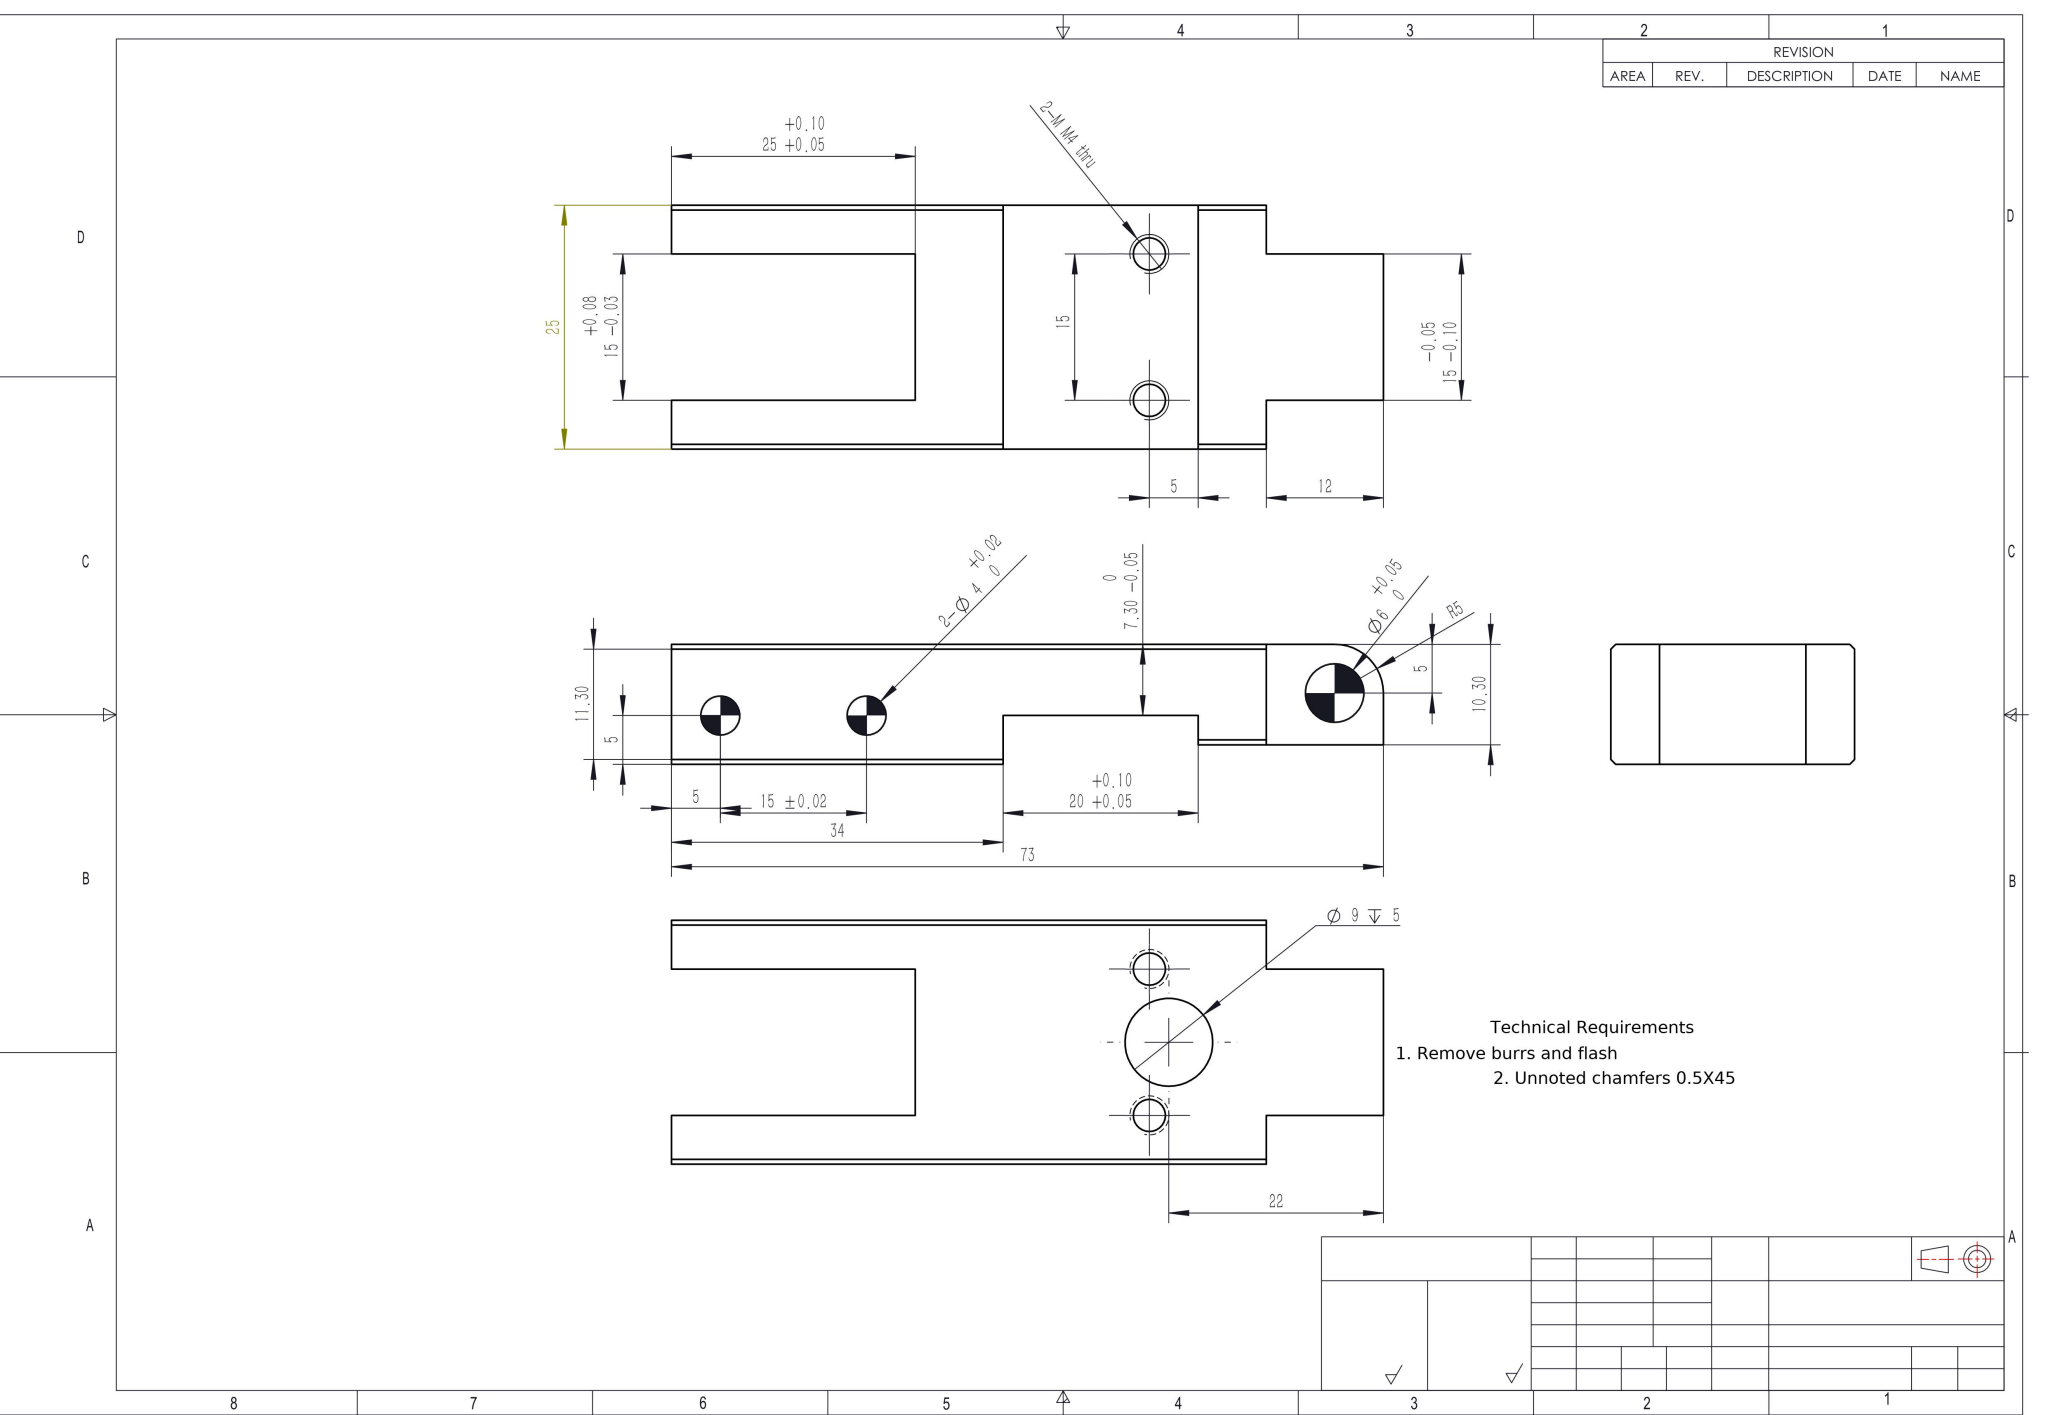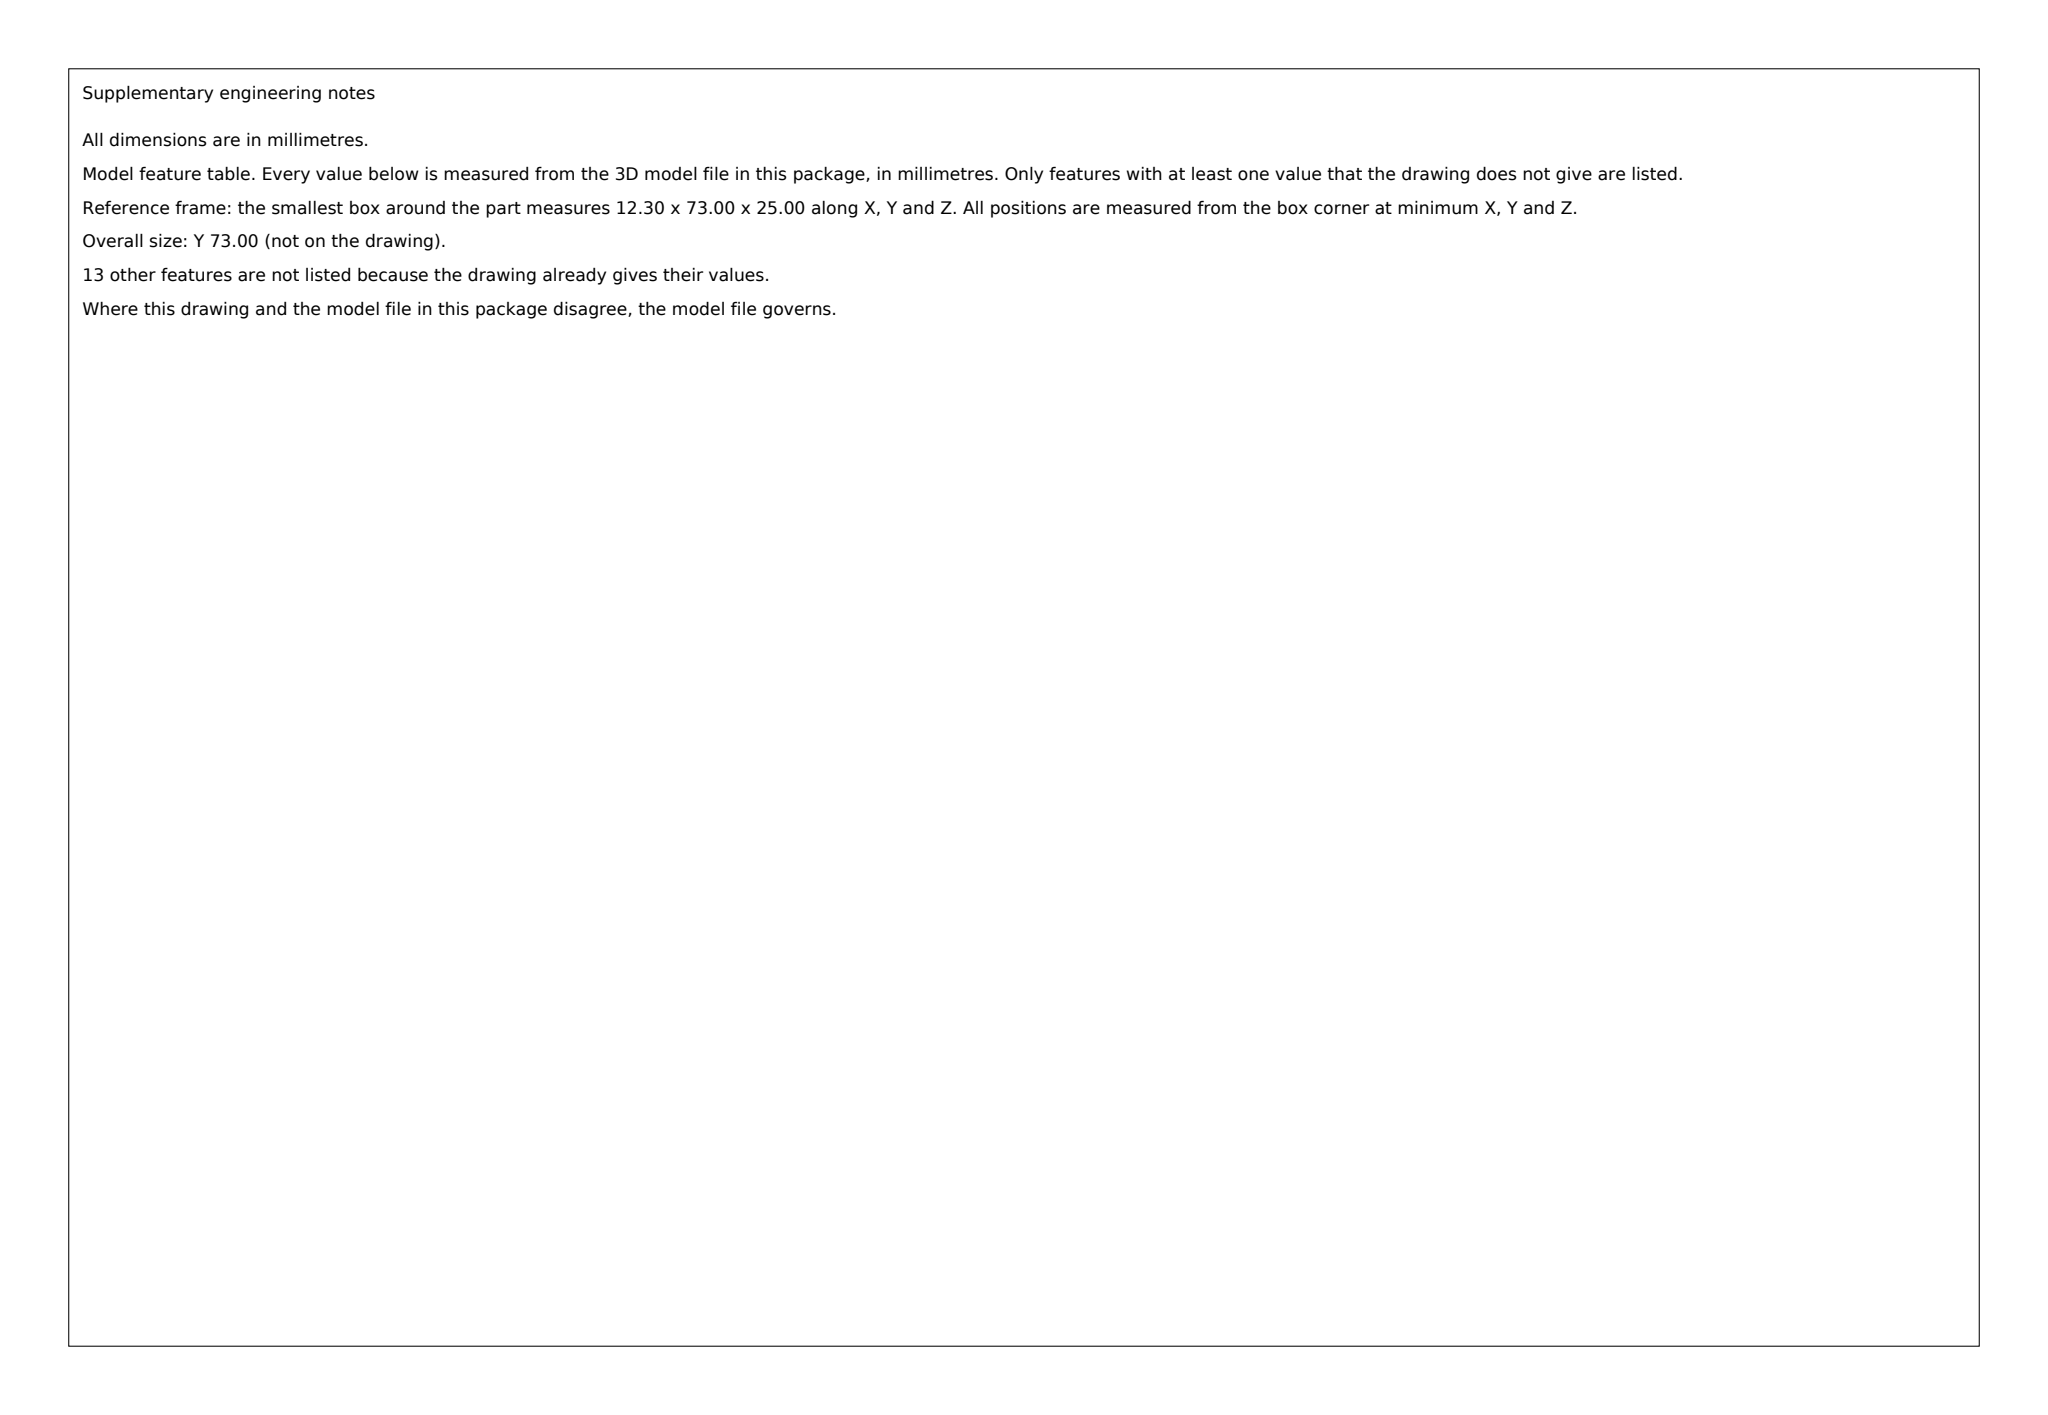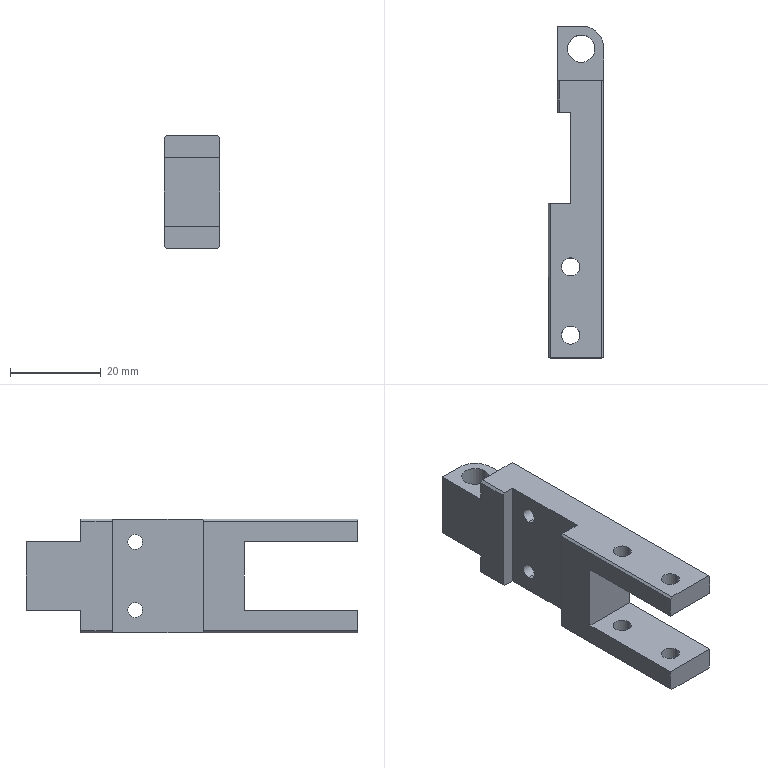Part | SolidWorks | mm | 1 solid | 42 faces | box 12.3 x 73 x 25 mm | volume 11925 mm3 | plane 25 | cylinder 17 | commonest cylinder face diameters 4 x8 3.3 x4 9 x2 6 x2 10 x1
build123d program:
from build123d import *

# Parameters (mm, degrees)
SKETCH1_W                    = 12.3
SKETCH1_H                    = 25
BOSS_EXTRUDE1_DEPTH          = 85
SKETCH2_W                    = 25
SKETCH2_H                    = 5
BOSS_EXTRUDE2_DEPTH          = 5
SKETCH4_W                    = 15
SKETCH4_H                    = 35
CUT_EXTRUDE1_DEPTH           = 87.79
SIZE_MM_DOWEL_HOLE_1_D       = 4
SKETCH7_W                    = 12.3
SKETCH7_H                    = 10
CUT_EXTRUDE2_DEPTH           = 90.299
SKETCH8_W                    = 5
SKETCH8_H                    = 20
CUT_EXTRUDE3_DEPTH           = 90.299
SKETCH14_W                   = 17.3
SKETCH14_H                   = 5
CUT_EXTRUDE4_DEPTH           = 90.299
SKETCH15_W                   = 12.3
SKETCH15_H                   = 5
CUT_EXTRUDE5_DEPTH           = 9
SKETCH22_W                   = 12.3
SKETCH22_H                   = 15
BOSS_EXTRUDE3_DEPTH          = 3
FILLET1_R                    = 5
SIZE_MM_DOWEL_HOLE_3_D       = 6
SIZE_MM_DOWEL_HOLE_3_DEPTH   = 35
CUT_EXTRUDE7_DEPTH           = 2
F_4_0_4_DIAMETER_HOLE1_D     = 9
F_4_0_4_DIAMETER_HOLE1_DEPTH = 5
M4_TAPPED_HOLE1_D            = 3.3
M4_TAPPED_HOLE1_DEPTH        = 11.5
M4_TAPPED_HOLE1_TIP          = 0.9914
CHAMFER1_SIZE                = 0.5


with BuildPart() as part:
    # Sketch1 → Boss-Extrude1 (new body)
    with BuildSketch(Plane(origin=(0, 0, 0), x_dir=(1, 0, 0), z_dir=(0, 1, 0))):
        Rectangle(SKETCH1_W, SKETCH1_H)
    extrude(amount=BOSS_EXTRUDE1_DEPTH)

    # Sketch2 → Boss-Extrude2 (add)
    with BuildSketch(Plane(origin=(6.15, 0, 0), x_dir=(0, 0, -1), z_dir=(1, 0, 0))):
        with Locations((0, 82.5)):
            Rectangle(SKETCH2_W, SKETCH2_H)
    extrude(amount=BOSS_EXTRUDE2_DEPTH)

    # Sketch4 → Cut-Extrude1 (cut, through all)
    with BuildSketch(Plane(origin=(6.15, 0, 0), x_dir=(0, 0, -1), z_dir=(1, 0, 0))):
        with Locations((0, 17.5)):
            Rectangle(SKETCH4_W, SKETCH4_H)
    extrude(amount=-CUT_EXTRUDE1_DEPTH, mode=Mode.SUBTRACT)

    # Size mm Dowel Hole 1 (through all)
    with Locations(Plane(origin=(0, 0, -12.5), x_dir=(-1, 0, 0), z_dir=(0, 0, -1))):
        with Locations((1.15, 30), (1.15, 15)):
            Hole(SIZE_MM_DOWEL_HOLE_1_D / 2)

    # Sketch7 → Cut-Extrude2 (cut, through all)
    with BuildSketch(Plane.XY.offset(12.5)):
        with Locations((0, 5)):
            Rectangle(SKETCH7_W, SKETCH7_H)
    extrude(amount=-CUT_EXTRUDE2_DEPTH, mode=Mode.SUBTRACT)

    # Sketch8 → Cut-Extrude3 (cut, through all)
    with BuildSketch(Plane(origin=(0, 0, -12.5), x_dir=(-1, 0, 0), z_dir=(0, 0, -1))):
        with Locations((3.65, 54)):
            Rectangle(SKETCH8_W, SKETCH8_H)
    extrude(amount=-CUT_EXTRUDE3_DEPTH, mode=Mode.SUBTRACT)

    # Sketch14 → Cut-Extrude4 (cut, through all)
    with BuildSketch(Plane(origin=(0, 0, -12.5), x_dir=(-1, 0, 0), z_dir=(0, 0, -1))):
        with Locations((-2.5, 82.5)):
            Rectangle(SKETCH14_W, SKETCH14_H)
    extrude(amount=-CUT_EXTRUDE4_DEPTH, mode=Mode.SUBTRACT)

    # Sketch15 → Cut-Extrude5 (cut)
    with BuildSketch(Plane(origin=(0, 80, 0), x_dir=(1, 0, 0), z_dir=(0, 1, 0))):
        with Locations((0, -10)):
            Rectangle(SKETCH15_W, SKETCH15_H)
        with Locations((0, 10)):
            Rectangle(SKETCH15_W, SKETCH15_H)
    extrude(amount=-CUT_EXTRUDE5_DEPTH, mode=Mode.SUBTRACT)

    # Sketch22 → Boss-Extrude3 (add)
    with BuildSketch(Plane(origin=(0, 80, 0), x_dir=(1, 0, 0), z_dir=(0, 1, 0))):
        Rectangle(SKETCH22_W, SKETCH22_H)
    extrude(amount=BOSS_EXTRUDE3_DEPTH)

    # Fillet1
    fillet1_edges = [part.edges().sort_by_distance(p)[0] for p in [
        (6.15, 83, 0),
    ]]
    fillet(fillet1_edges, radius=FILLET1_R)

    # Size mm Dowel Hole 3
    with Locations(Plane(origin=(0, 0, -7.5), x_dir=(-1, 0, 0), z_dir=(0, 0, -1))):
        with Locations((-1.15, 78)):
            Hole(SIZE_MM_DOWEL_HOLE_3_D / 2, depth=SIZE_MM_DOWEL_HOLE_3_DEPTH)

    # Sketch19 → Cut-Extrude7 (cut)
    with BuildSketch(Plane.ZY.offset(6.15)):
        Polygon((7.5, 83), (-7.5, 83), (-7.5, 71), (-12.5, 71), (-12.5, 64), (12.5, 64), (12.5, 71), (7.5, 71), align=None)
    extrude(amount=-CUT_EXTRUDE7_DEPTH, mode=Mode.SUBTRACT)

    # 4.0 _4_ Diameter Hole1
    with Locations(Plane(origin=(6.15, 0, 0), x_dir=(0, 0, -1), z_dir=(1, 0, 0))):
        with Locations((0, 61)):
            Hole(F_4_0_4_DIAMETER_HOLE1_D / 2, depth=F_4_0_4_DIAMETER_HOLE1_DEPTH)

    # M4 Tapped Hole1
    with Locations(Plane.ZY.offset(1.15)):
        with Locations((-7.5, 59), (7.5, 59)):
            Hole(M4_TAPPED_HOLE1_D / 2, depth=M4_TAPPED_HOLE1_DEPTH)
            with Locations((0, 0, -(M4_TAPPED_HOLE1_DEPTH + M4_TAPPED_HOLE1_TIP / 2))):  # 118° drill point
                Cone(0, M4_TAPPED_HOLE1_D / 2, M4_TAPPED_HOLE1_TIP, mode=Mode.SUBTRACT)

    # Chamfer1
    chamfer1_edges = [part.edges().sort_by_distance(p)[0] for p in [
        (6.15, 40.5, 12.5),
        (6.15, 40.5, -12.5),
        (-4.15, 67.5, 12.5),
        (-4.15, 67.5, -12.5),
        (-6.15, 27, 12.5),
        (-6.15, 27, -12.5),
    ]]
    chamfer(chamfer1_edges, length=CHAMFER1_SIZE)


solid = part.part